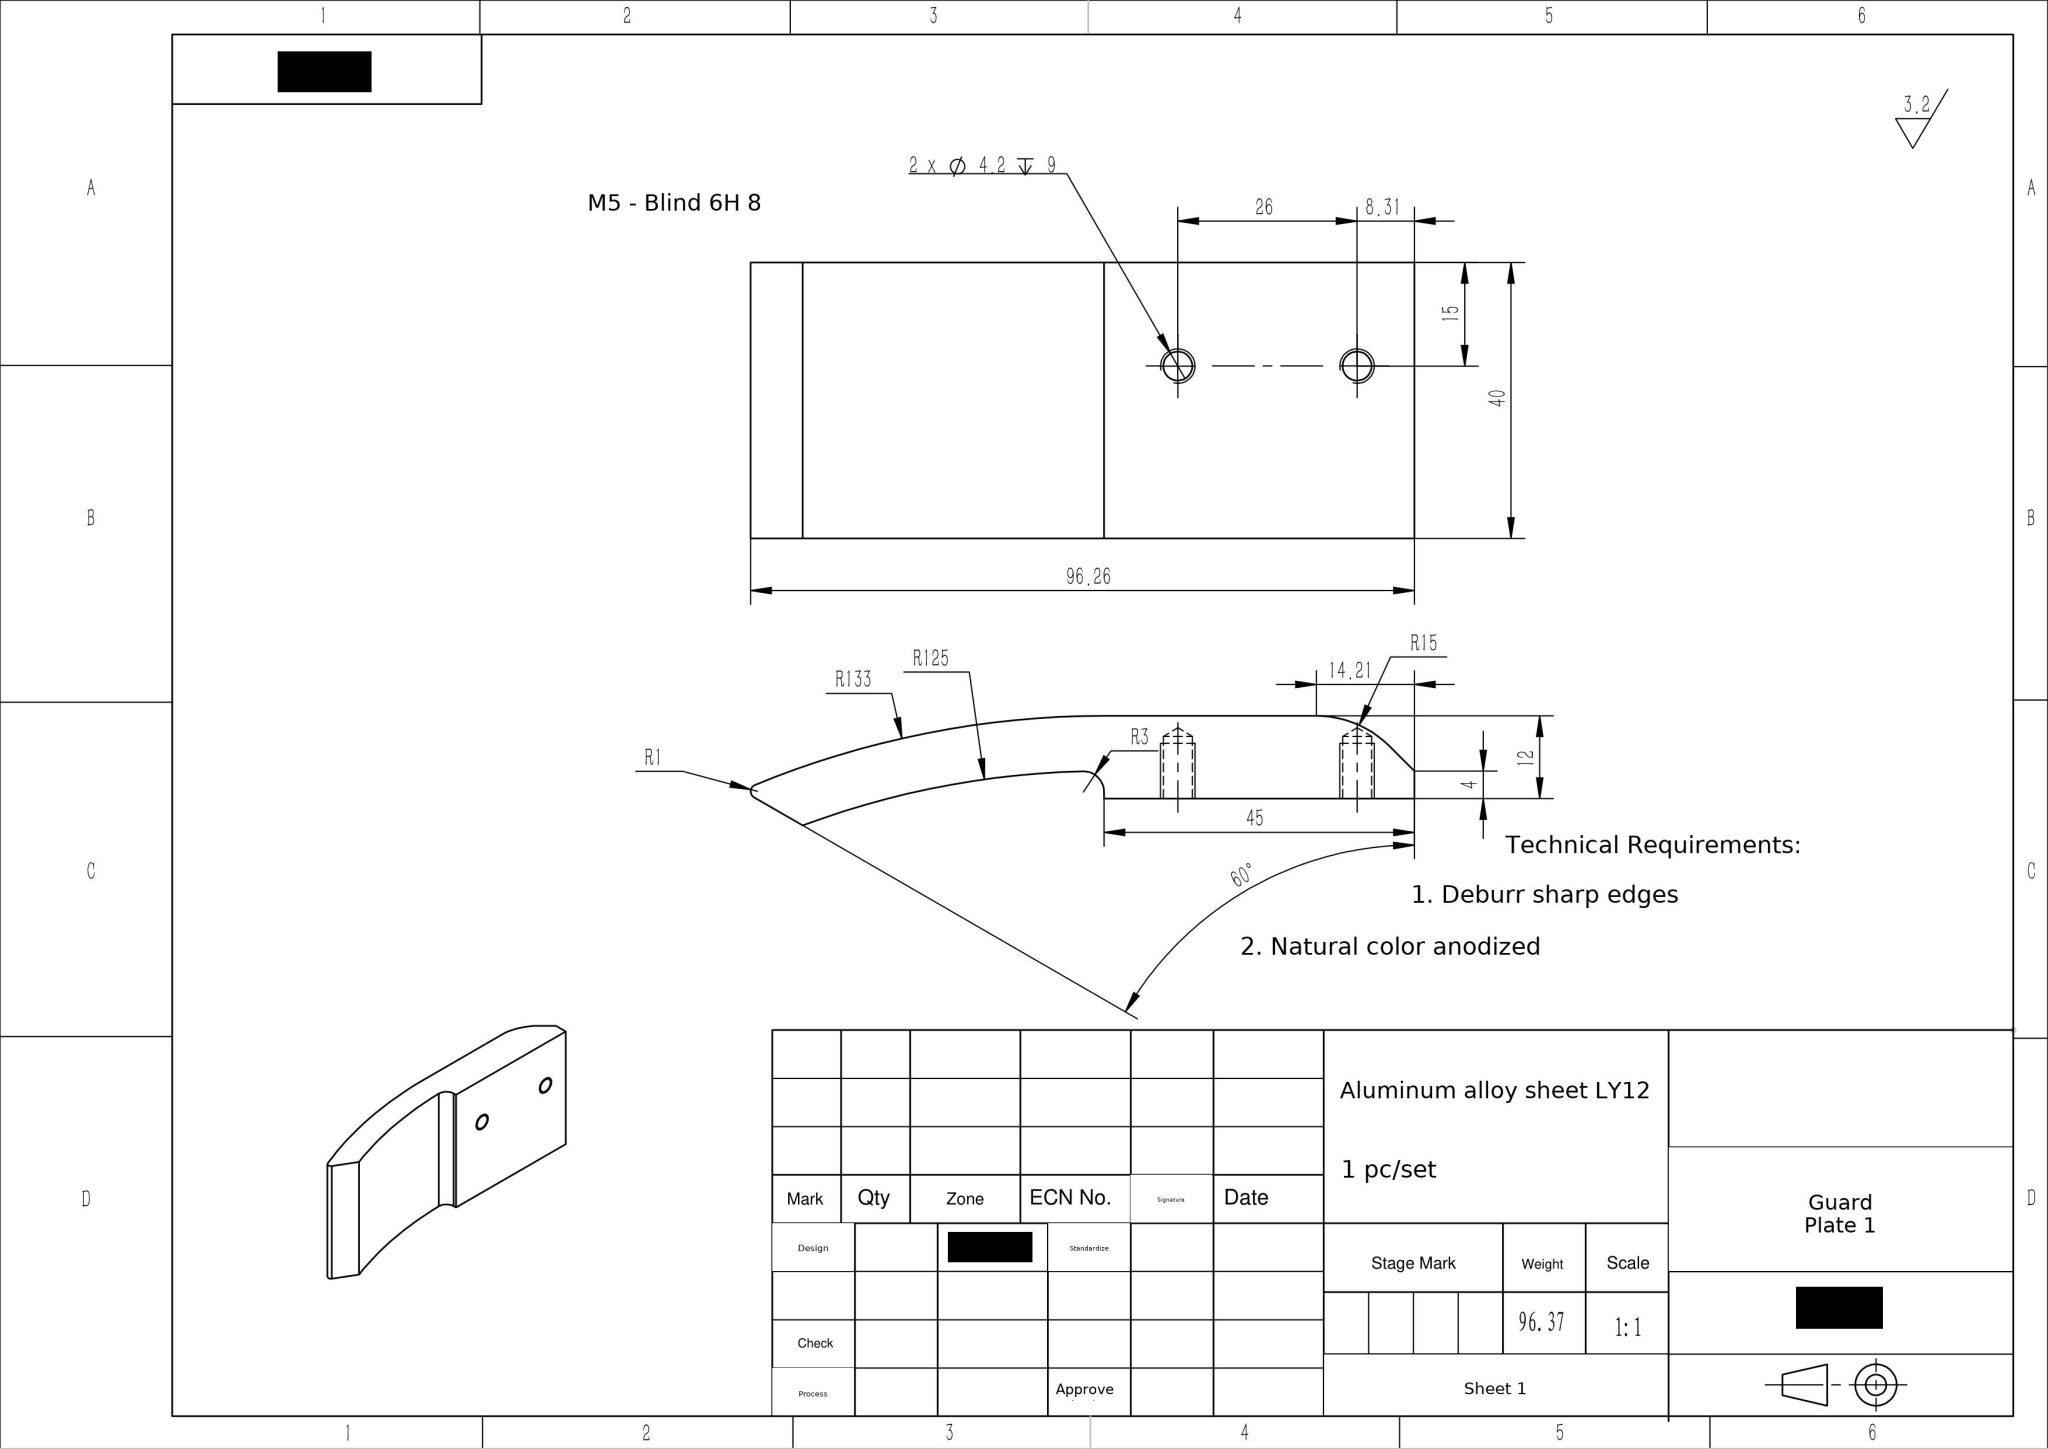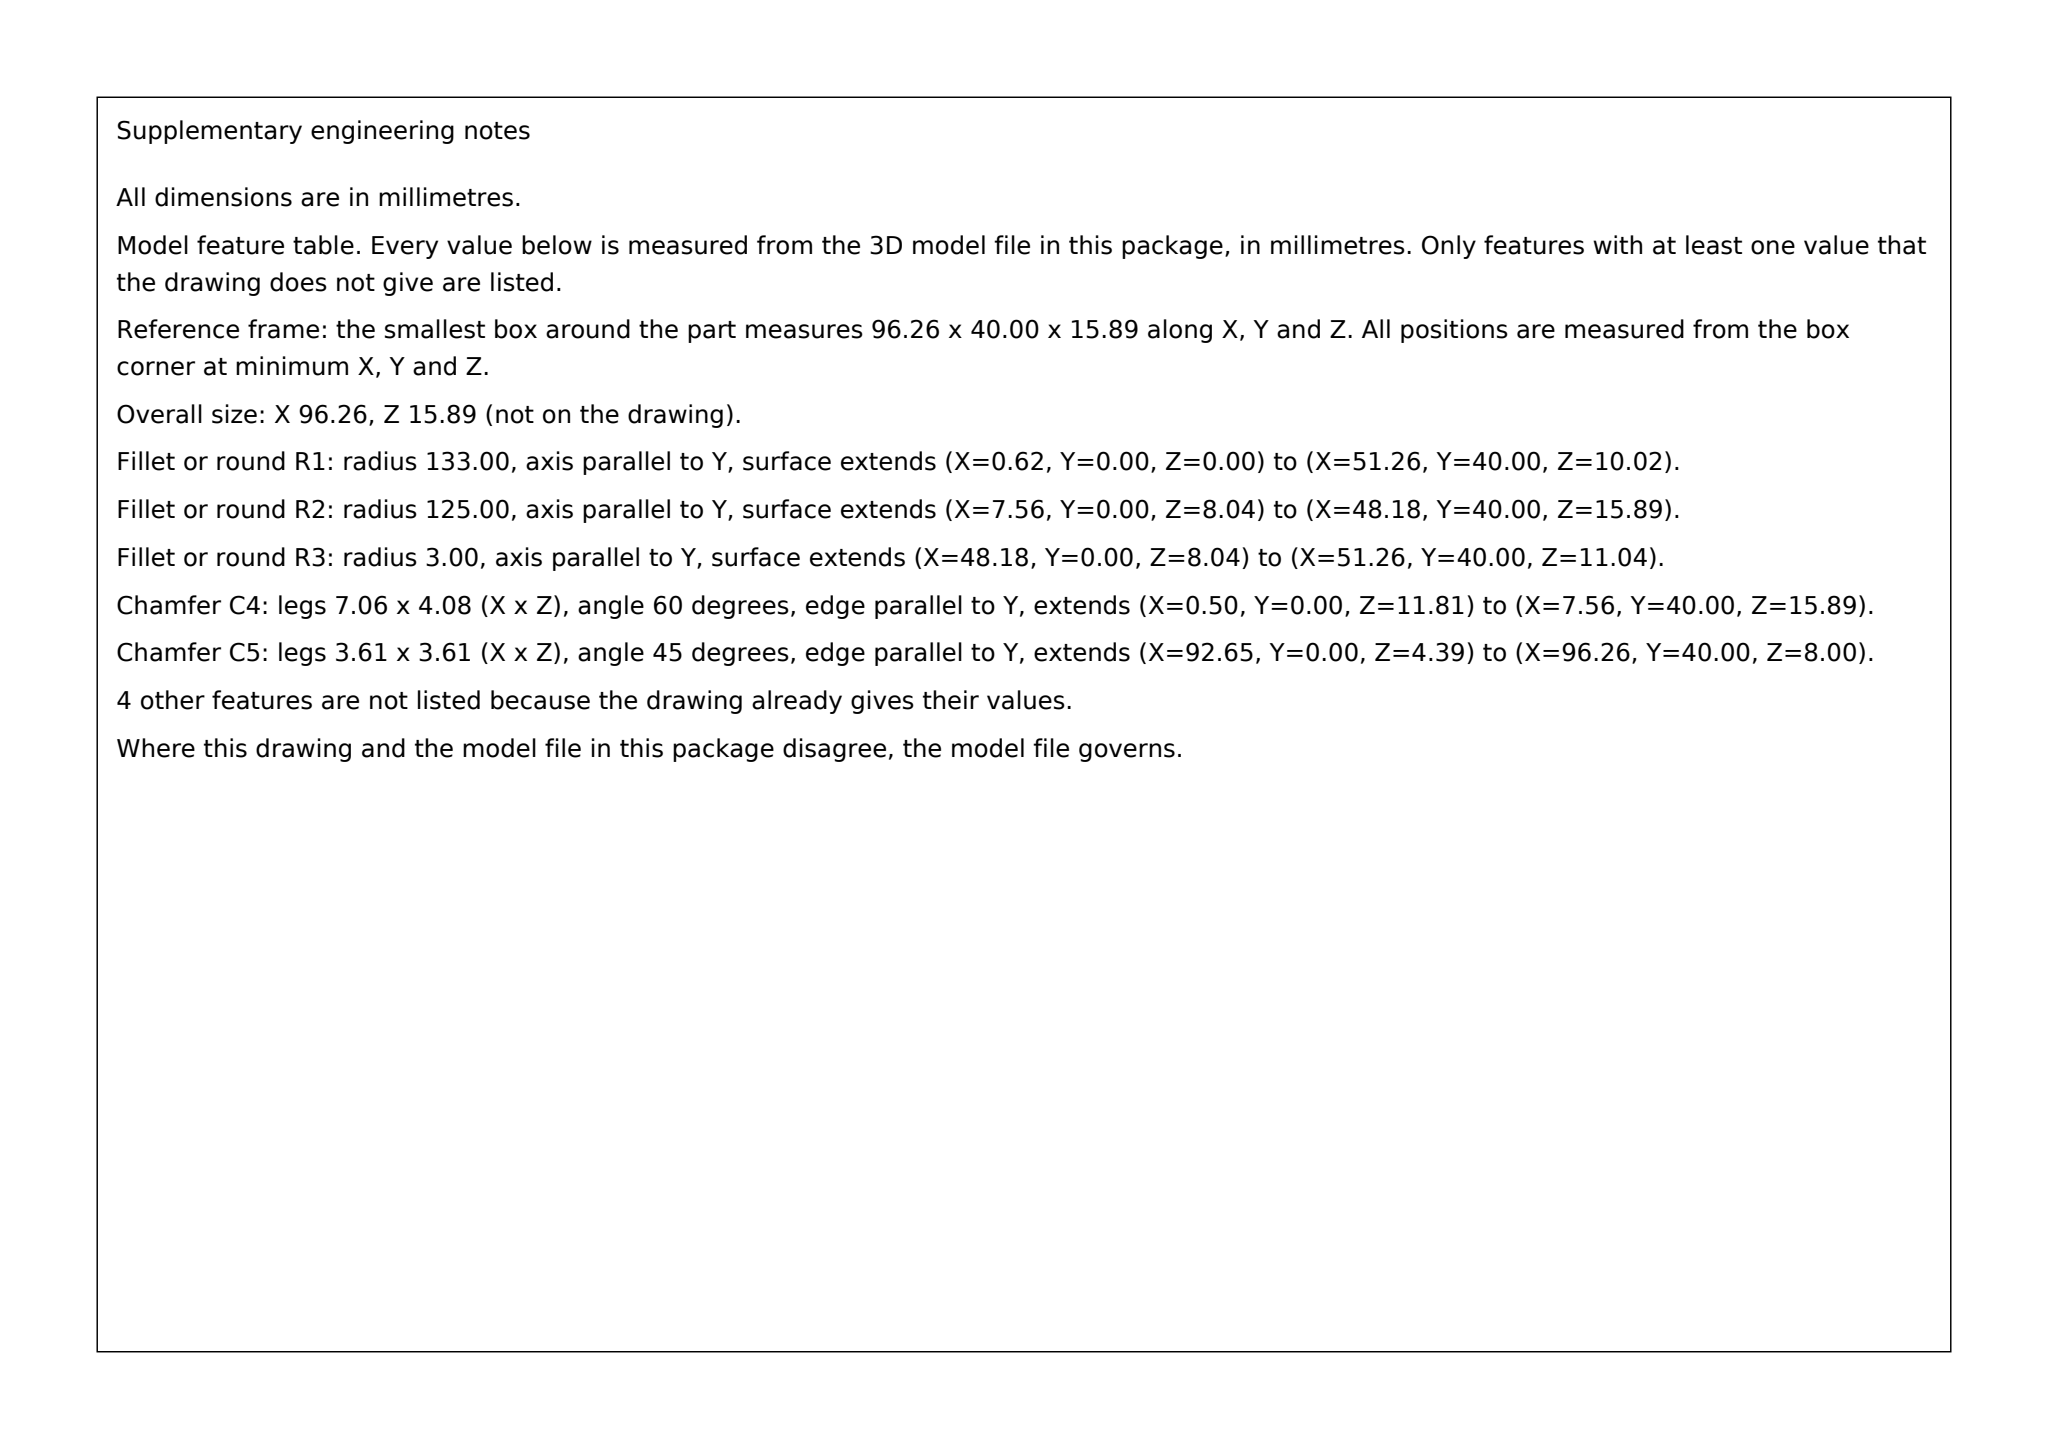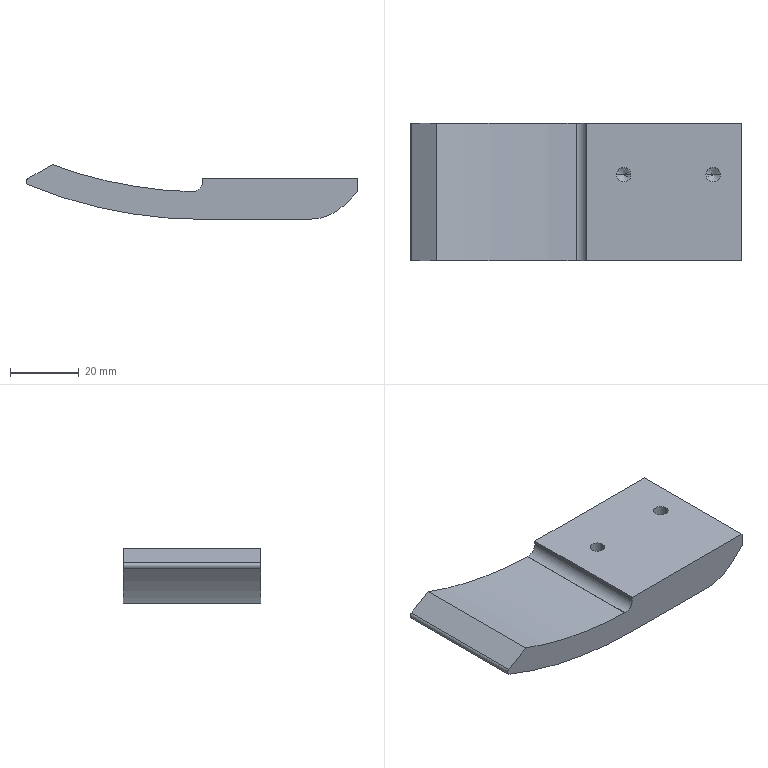Part | SolidWorks | mm | material Aluminum alloy sheet LY12 | 1 solid | 22 faces | box 96.26 x 40 x 15.89 mm | volume 35692 mm3 | cylinder 10 | plane 8 | cone 4 | commonest cylinder face diameters 4.2 x4 6 x2 250 x1 266 x1 30 x1 2 x1
build123d program:
from build123d import *

# Parameters (mm, degrees)
BOSS_EXTRUDE1_DEPTH   = 40
SKETCH5_W             = 45
SKETCH5_H             = 40
BOSS_EXTRUDE2_DEPTH   = 4
M5_TAPPED_HOLE1_D     = 4.2
M5_TAPPED_HOLE1_DEPTH = 9
M5_TAPPED_HOLE1_TIP   = 1.262
CHAMFER1_SIZE         = 8
FILLET1_R             = 15
FILLET2_R             = 1
FILLET3_R             = 3


with BuildPart() as part:
    # Sketch1 → Boss-Extrude1 (new body)
    with BuildSketch(Plane(origin=(0, 0, 0), x_dir=(1, 0, 0), z_dir=(0, 1, 0))):
        with BuildLine():
            Line((0, 0), (45, 0))
            Line((45, 0), (45, -8))
            Line((45, -8), (0, -8))
            ThreePointArc((0, -8), (-22.199, -9.987), (-43.693, -15.885))
            Line((-43.693, -15.885), (-52.5, -10.8))
            ThreePointArc((-52.5, -10.8), (-26.8, -2.728), (0, 0))
        make_face()
    extrude(amount=BOSS_EXTRUDE1_DEPTH)

    # Sketch5 → Boss-Extrude2 (add)
    with BuildSketch(Plane.XY.offset(8)):
        with Locations((22.5, 20)):
            Rectangle(SKETCH5_W, SKETCH5_H)
    extrude(amount=BOSS_EXTRUDE2_DEPTH)

    # M5 Tapped Hole1
    with Locations(Plane.XY.offset(12)):
        with Locations((36.695, 25), (10.695, 25)):
            Hole(M5_TAPPED_HOLE1_D / 2, depth=M5_TAPPED_HOLE1_DEPTH)
            with Locations((0, 0, -(M5_TAPPED_HOLE1_DEPTH + M5_TAPPED_HOLE1_TIP / 2))):  # 118° drill point
                Cone(0, M5_TAPPED_HOLE1_D / 2, M5_TAPPED_HOLE1_TIP, mode=Mode.SUBTRACT)

    # Chamfer1
    chamfer1_edges = [part.edges().sort_by_distance(p)[0] for p in [
        (45, 20, 0),
    ]]
    chamfer(chamfer1_edges, length=CHAMFER1_SIZE)

    # Fillet1
    fillet1_edges = [part.edges().sort_by_distance(p)[0] for p in [
        (37, 20, 0),
    ]]
    fillet(fillet1_edges, radius=FILLET1_R)

    # Fillet2
    fillet2_edges = [part.edges().sort_by_distance(p)[0] for p in [
        (-52.5, 20, 10.8),
    ]]
    fillet(fillet2_edges, radius=FILLET2_R)

    # Fillet3
    fillet3_edges = [part.edges().sort_by_distance(p)[0] for p in [
        (0, 20, 8),
    ]]
    fillet(fillet3_edges, radius=FILLET3_R)


solid = part.part
STEP:
#1=CARTESIAN_POINT('',(-3.,40.,8.037));
#2=VERTEX_POINT('',#1);
#3=CARTESIAN_POINT('',(0.,40.,11.037));
#4=VERTEX_POINT('',#3);
#5=CARTESIAN_POINT('',(-3.,40.,11.037));
#6=DIRECTION('',(0.,-1.,0.));
#7=DIRECTION('',(0.,0.,1.));
#8=AXIS2_PLACEMENT_3D('',#5,#6,#7);
#9=CIRCLE('',#8,3.);
#10=EDGE_CURVE('',#2,#4,#9,.T.);
#11=ORIENTED_EDGE('',*,*,#10,.F.);
#12=CARTESIAN_POINT('',(-3.,0.,8.037));
#13=VERTEX_POINT('',#12);
#14=CARTESIAN_POINT('',(-3.,40.,8.037));
#15=DIRECTION('',(0.,-1.,0.));
#16=VECTOR('',#15,1000.);
#17=LINE('',#14,#16);
#18=EDGE_CURVE('',#2,#13,#17,.T.);
#19=ORIENTED_EDGE('',*,*,#18,.T.);
#20=CARTESIAN_POINT('',(-0.,0.,11.037));
#21=VERTEX_POINT('',#20);
#22=CARTESIAN_POINT('',(-3.,0.,11.037));
#23=DIRECTION('',(0.,1.,0.));
#24=DIRECTION('',(0.,0.,1.));
#25=AXIS2_PLACEMENT_3D('',#22,#23,#24);
#26=CIRCLE('',#25,3.);
#27=EDGE_CURVE('',#21,#13,#26,.T.);
#28=ORIENTED_EDGE('',*,*,#27,.F.);
#29=CARTESIAN_POINT('',(-0.,-0.,11.037));
#30=DIRECTION('',(-0.,-1.,0.));
#31=VECTOR('',#30,1000.);
#32=LINE('',#29,#31);
#33=EDGE_CURVE('',#4,#21,#32,.T.);
#34=ORIENTED_EDGE('',*,*,#33,.F.);
#35=EDGE_LOOP('',(#11,#19,#28,#34));
#36=FACE_OUTER_BOUND('',#35,.T.);
#37=CARTESIAN_POINT('',(-3.,40.,11.037));
#38=DIRECTION('',(0.,-1.,0.));
#39=DIRECTION('',(0.,0.,-1.));
#40=AXIS2_PLACEMENT_3D('',#37,#38,#39);
#41=CYLINDRICAL_SURFACE('',#40,3.);
#42=ADVANCED_FACE('',(#36),#41,.F.);
#43=CARTESIAN_POINT('',(34.595,25.,3.));
#44=VERTEX_POINT('',#43);
#45=CARTESIAN_POINT('',(38.795,25.,3.));
#46=VERTEX_POINT('',#45);
#47=CARTESIAN_POINT('',(36.695,25.,3.));
#48=DIRECTION('',(0.,0.,1.));
#49=DIRECTION('',(1.,0.,0.));
#50=AXIS2_PLACEMENT_3D('',#47,#48,#49);
#51=CIRCLE('',#50,2.1);
#52=EDGE_CURVE('',#44,#46,#51,.T.);
#53=ORIENTED_EDGE('',*,*,#52,.F.);
#54=CARTESIAN_POINT('',(34.595,25.,12.));
#55=VERTEX_POINT('',#54);
#56=CARTESIAN_POINT('',(34.595,25.,12.));
#57=DIRECTION('',(0.,0.,1.));
#58=VECTOR('',#57,1000.);
#59=LINE('',#56,#58);
#60=EDGE_CURVE('',#44,#55,#59,.T.);
#61=ORIENTED_EDGE('',*,*,#60,.T.);
#62=CARTESIAN_POINT('',(38.795,25.,12.));
#63=VERTEX_POINT('',#62);
#64=CARTESIAN_POINT('',(36.695,25.,12.));
#65=DIRECTION('',(0.,0.,1.));
#66=DIRECTION('',(1.,0.,0.));
#67=AXIS2_PLACEMENT_3D('',#64,#65,#66);
#68=CIRCLE('',#67,2.1);
#69=EDGE_CURVE('',#55,#63,#68,.T.);
#70=ORIENTED_EDGE('',*,*,#69,.T.);
#71=CARTESIAN_POINT('',(38.795,25.,12.));
#72=DIRECTION('',(0.,0.,1.));
#73=VECTOR('',#72,1000.);
#74=LINE('',#71,#73);
#75=EDGE_CURVE('',#46,#63,#74,.T.);
#76=ORIENTED_EDGE('',*,*,#75,.F.);
#77=EDGE_LOOP('',(#53,#61,#70,#76));
#78=FACE_OUTER_BOUND('',#77,.T.);
#79=CARTESIAN_POINT('',(36.695,25.,12.));
#80=DIRECTION('',(0.,0.,1.));
#81=DIRECTION('',(1.,0.,0.));
#82=AXIS2_PLACEMENT_3D('',#79,#80,#81);
#83=CYLINDRICAL_SURFACE('',#82,2.1);
#84=ADVANCED_FACE('',(#78),#83,.F.);
#85=CARTESIAN_POINT('',(36.695,25.,1.738));
#86=VERTEX_POINT('',#85);
#87=CARTESIAN_POINT('',(38.795,25.,3.));
#88=DIRECTION('',(0.8572,0.,0.515));
#89=VECTOR('',#88,1000.);
#90=LINE('',#87,#89);
#91=EDGE_CURVE('',#86,#46,#90,.T.);
#92=ORIENTED_EDGE('',*,*,#91,.F.);
#93=CARTESIAN_POINT('',(34.595,25.,3.));
#94=DIRECTION('',(-0.8572,0.,0.515));
#95=VECTOR('',#94,1000.);
#96=LINE('',#93,#95);
#97=EDGE_CURVE('',#86,#44,#96,.T.);
#98=ORIENTED_EDGE('',*,*,#97,.T.);
#99=ORIENTED_EDGE('',*,*,#52,.T.);
#100=EDGE_LOOP('',(#92,#98,#99));
#101=FACE_OUTER_BOUND('',#100,.T.);
#102=CARTESIAN_POINT('',(36.695,25.,3.));
#103=DIRECTION('',(0.,0.,1.));
#104=DIRECTION('',(1.,0.,0.));
#105=AXIS2_PLACEMENT_3D('',#102,#103,#104);
#106=CONICAL_SURFACE('',#105,2.1,1.03);
#107=ADVANCED_FACE('',(#101),#106,.F.);
#108=CARTESIAN_POINT('',(8.595,25.,3.));
#109=VERTEX_POINT('',#108);
#110=CARTESIAN_POINT('',(12.795,25.,3.));
#111=VERTEX_POINT('',#110);
#112=CARTESIAN_POINT('',(10.695,25.,3.));
#113=DIRECTION('',(0.,0.,1.));
#114=DIRECTION('',(1.,0.,0.));
#115=AXIS2_PLACEMENT_3D('',#112,#113,#114);
#116=CIRCLE('',#115,2.1);
#117=EDGE_CURVE('',#109,#111,#116,.T.);
#118=ORIENTED_EDGE('',*,*,#117,.F.);
#119=CARTESIAN_POINT('',(8.595,25.,12.));
#120=VERTEX_POINT('',#119);
#121=CARTESIAN_POINT('',(8.595,25.,12.));
#122=DIRECTION('',(0.,0.,1.));
#123=VECTOR('',#122,1000.);
#124=LINE('',#121,#123);
#125=EDGE_CURVE('',#109,#120,#124,.T.);
#126=ORIENTED_EDGE('',*,*,#125,.T.);
#127=CARTESIAN_POINT('',(12.795,25.,12.));
#128=VERTEX_POINT('',#127);
#129=CARTESIAN_POINT('',(10.695,25.,12.));
#130=DIRECTION('',(0.,0.,1.));
#131=DIRECTION('',(1.,0.,0.));
#132=AXIS2_PLACEMENT_3D('',#129,#130,#131);
#133=CIRCLE('',#132,2.1);
#134=EDGE_CURVE('',#120,#128,#133,.T.);
#135=ORIENTED_EDGE('',*,*,#134,.T.);
#136=CARTESIAN_POINT('',(12.795,25.,12.));
#137=DIRECTION('',(0.,0.,1.));
#138=VECTOR('',#137,1000.);
#139=LINE('',#136,#138);
#140=EDGE_CURVE('',#111,#128,#139,.T.);
#141=ORIENTED_EDGE('',*,*,#140,.F.);
#142=EDGE_LOOP('',(#118,#126,#135,#141));
#143=FACE_OUTER_BOUND('',#142,.T.);
#144=CARTESIAN_POINT('',(10.695,25.,12.));
#145=DIRECTION('',(0.,0.,1.));
#146=DIRECTION('',(1.,0.,0.));
#147=AXIS2_PLACEMENT_3D('',#144,#145,#146);
#148=CYLINDRICAL_SURFACE('',#147,2.1);
#149=ADVANCED_FACE('',(#143),#148,.F.);
#150=CARTESIAN_POINT('',(10.695,25.,1.738));
#151=VERTEX_POINT('',#150);
#152=CARTESIAN_POINT('',(12.795,25.,3.));
#153=DIRECTION('',(0.8572,0.,0.515));
#154=VECTOR('',#153,1000.);
#155=LINE('',#152,#154);
#156=EDGE_CURVE('',#151,#111,#155,.T.);
#157=ORIENTED_EDGE('',*,*,#156,.F.);
#158=CARTESIAN_POINT('',(8.595,25.,3.));
#159=DIRECTION('',(-0.8572,0.,0.515));
#160=VECTOR('',#159,1000.);
#161=LINE('',#158,#160);
#162=EDGE_CURVE('',#151,#109,#161,.T.);
#163=ORIENTED_EDGE('',*,*,#162,.T.);
#164=ORIENTED_EDGE('',*,*,#117,.T.);
#165=EDGE_LOOP('',(#157,#163,#164));
#166=FACE_OUTER_BOUND('',#165,.T.);
#167=CARTESIAN_POINT('',(10.695,25.,3.));
#168=DIRECTION('',(0.,0.,1.));
#169=DIRECTION('',(1.,0.,0.));
#170=AXIS2_PLACEMENT_3D('',#167,#168,#169);
#171=CONICAL_SURFACE('',#170,2.1,1.03);
#172=ADVANCED_FACE('',(#166),#171,.F.);
#173=CARTESIAN_POINT('',(-43.693,0.,15.885));
#174=VERTEX_POINT('',#173);
#175=CARTESIAN_POINT('',(-3.074,0.,8.038));
#176=VERTEX_POINT('',#175);
#177=CARTESIAN_POINT('',(0.,0.,133.));
#178=DIRECTION('',(0.,-1.,0.));
#179=DIRECTION('',(0.,0.,1.));
#180=AXIS2_PLACEMENT_3D('',#177,#178,#179);
#181=CIRCLE('',#180,125.);
#182=EDGE_CURVE('',#174,#176,#181,.T.);
#183=ORIENTED_EDGE('',*,*,#182,.T.);
#184=CARTESIAN_POINT('',(-3.074,40.,8.038));
#185=VERTEX_POINT('',#184);
#186=CARTESIAN_POINT('',(-3.074,40.,8.038));
#187=DIRECTION('',(0.,1.,0.));
#188=VECTOR('',#187,1000.);
#189=LINE('',#186,#188);
#190=EDGE_CURVE('',#176,#185,#189,.T.);
#191=ORIENTED_EDGE('',*,*,#190,.T.);
#192=CARTESIAN_POINT('',(-43.693,40.,15.885));
#193=VERTEX_POINT('',#192);
#194=CARTESIAN_POINT('',(0.,40.,133.));
#195=DIRECTION('',(0.,-1.,0.));
#196=DIRECTION('',(0.,0.,1.));
#197=AXIS2_PLACEMENT_3D('',#194,#195,#196);
#198=CIRCLE('',#197,125.);
#199=EDGE_CURVE('',#193,#185,#198,.T.);
#200=ORIENTED_EDGE('',*,*,#199,.F.);
#201=CARTESIAN_POINT('',(-43.693,40.,15.885));
#202=DIRECTION('',(0.,-1.,0.));
#203=VECTOR('',#202,1000.);
#204=LINE('',#201,#203);
#205=EDGE_CURVE('',#193,#174,#204,.T.);
#206=ORIENTED_EDGE('',*,*,#205,.T.);
#207=EDGE_LOOP('',(#183,#191,#200,#206));
#208=FACE_OUTER_BOUND('',#207,.T.);
#209=CARTESIAN_POINT('',(0.,40.,133.));
#210=DIRECTION('',(0.,-1.,0.));
#211=DIRECTION('',(0.,0.,-1.));
#212=AXIS2_PLACEMENT_3D('',#209,#210,#211);
#213=CYLINDRICAL_SURFACE('',#212,125.);
#214=ADVANCED_FACE('',(#208),#213,.F.);
#215=CARTESIAN_POINT('',(45.,-0.,12.));
#216=VERTEX_POINT('',#215);
#217=CARTESIAN_POINT('',(45.,0.,8.));
#218=VERTEX_POINT('',#217);
#219=CARTESIAN_POINT('',(45.,0.,0.));
#220=DIRECTION('',(0.,0.,-1.));
#221=VECTOR('',#220,1000.);
#222=LINE('',#219,#221);
#223=EDGE_CURVE('',#216,#218,#222,.T.);
#224=ORIENTED_EDGE('',*,*,#223,.T.);
#225=CARTESIAN_POINT('',(45.,40.,8.));
#226=VERTEX_POINT('',#225);
#227=CARTESIAN_POINT('',(45.,40.,8.));
#228=DIRECTION('',(0.,1.,0.));
#229=VECTOR('',#228,1000.);
#230=LINE('',#227,#229);
#231=EDGE_CURVE('',#218,#226,#230,.T.);
#232=ORIENTED_EDGE('',*,*,#231,.T.);
#233=CARTESIAN_POINT('',(45.,40.,12.));
#234=VERTEX_POINT('',#233);
#235=CARTESIAN_POINT('',(45.,40.,0.));
#236=DIRECTION('',(0.,0.,-1.));
#237=VECTOR('',#236,1000.);
#238=LINE('',#235,#237);
#239=EDGE_CURVE('',#234,#226,#238,.T.);
#240=ORIENTED_EDGE('',*,*,#239,.F.);
#241=CARTESIAN_POINT('',(45.,40.,12.));
#242=DIRECTION('',(-0.,1.,0.));
#243=VECTOR('',#242,1000.);
#244=LINE('',#241,#243);
#245=EDGE_CURVE('',#216,#234,#244,.T.);
#246=ORIENTED_EDGE('',*,*,#245,.F.);
#247=EDGE_LOOP('',(#224,#232,#240,#246));
#248=FACE_OUTER_BOUND('',#247,.T.);
#249=CARTESIAN_POINT('',(45.,40.,0.));
#250=DIRECTION('',(-1.,0.,0.));
#251=DIRECTION('',(0.,0.,1.));
#252=AXIS2_PLACEMENT_3D('',#249,#250,#251);
#253=PLANE('',#252);
#254=ADVANCED_FACE('',(#248),#253,.F.);
#255=CARTESIAN_POINT('',(30.787,40.,0.));
#256=VERTEX_POINT('',#255);
#257=CARTESIAN_POINT('',(0.,40.,0.));
#258=VERTEX_POINT('',#257);
#259=CARTESIAN_POINT('',(0.,40.,0.));
#260=DIRECTION('',(-1.,0.,0.));
#261=VECTOR('',#260,1000.);
#262=LINE('',#259,#261);
#263=EDGE_CURVE('',#256,#258,#262,.T.);
#264=ORIENTED_EDGE('',*,*,#263,.F.);
#265=CARTESIAN_POINT('',(30.787,0.,0.));
#266=VERTEX_POINT('',#265);
#267=CARTESIAN_POINT('',(30.787,0.,0.));
#268=DIRECTION('',(0.,-1.,0.));
#269=VECTOR('',#268,1000.);
#270=LINE('',#267,#269);
#271=EDGE_CURVE('',#256,#266,#270,.T.);
#272=ORIENTED_EDGE('',*,*,#271,.T.);
#273=CARTESIAN_POINT('',(0.,0.,0.));
#274=VERTEX_POINT('',#273);
#275=CARTESIAN_POINT('',(0.,0.,0.));
#276=DIRECTION('',(-1.,0.,0.));
#277=VECTOR('',#276,1000.);
#278=LINE('',#275,#277);
#279=EDGE_CURVE('',#266,#274,#278,.T.);
#280=ORIENTED_EDGE('',*,*,#279,.T.);
#281=CARTESIAN_POINT('',(0.,40.,0.));
#282=DIRECTION('',(0.,-1.,0.));
#283=VECTOR('',#282,1000.);
#284=LINE('',#281,#283);
#285=EDGE_CURVE('',#258,#274,#284,.T.);
#286=ORIENTED_EDGE('',*,*,#285,.F.);
#287=EDGE_LOOP('',(#264,#272,#280,#286));
#288=FACE_OUTER_BOUND('',#287,.T.);
#289=CARTESIAN_POINT('',(0.,40.,0.));
#290=DIRECTION('',(0.,0.,1.));
#291=DIRECTION('',(1.,0.,0.));
#292=AXIS2_PLACEMENT_3D('',#289,#290,#291);
#293=PLANE('',#292);
#294=ADVANCED_FACE('',(#288),#293,.F.);
#295=CARTESIAN_POINT('',(-50.637,0.,10.017));
#296=VERTEX_POINT('',#295);
#297=CARTESIAN_POINT('',(0.,0.,133.));
#298=DIRECTION('',(0.,1.,0.));
#299=DIRECTION('',(0.,0.,1.));
#300=AXIS2_PLACEMENT_3D('',#297,#298,#299);
#301=CIRCLE('',#300,133.);
#302=EDGE_CURVE('',#274,#296,#301,.T.);
#303=ORIENTED_EDGE('',*,*,#302,.T.);
#304=CARTESIAN_POINT('',(-50.637,40.,10.017));
#305=VERTEX_POINT('',#304);
#306=CARTESIAN_POINT('',(-50.637,40.,10.017));
#307=DIRECTION('',(0.,1.,0.));
#308=VECTOR('',#307,1000.);
#309=LINE('',#306,#308);
#310=EDGE_CURVE('',#296,#305,#309,.T.);
#311=ORIENTED_EDGE('',*,*,#310,.T.);
#312=CARTESIAN_POINT('',(0.,40.,133.));
#313=DIRECTION('',(0.,1.,0.));
#314=DIRECTION('',(0.,0.,1.));
#315=AXIS2_PLACEMENT_3D('',#312,#313,#314);
#316=CIRCLE('',#315,133.);
#317=EDGE_CURVE('',#258,#305,#316,.T.);
#318=ORIENTED_EDGE('',*,*,#317,.F.);
#319=ORIENTED_EDGE('',*,*,#285,.T.);
#320=EDGE_LOOP('',(#303,#311,#318,#319));
#321=FACE_OUTER_BOUND('',#320,.T.);
#322=CARTESIAN_POINT('',(0.,40.,133.));
#323=DIRECTION('',(0.,-1.,0.));
#324=DIRECTION('',(0.,0.,-1.));
#325=AXIS2_PLACEMENT_3D('',#322,#323,#324);
#326=CYLINDRICAL_SURFACE('',#325,133.);
#327=ADVANCED_FACE('',(#321),#326,.T.);
#328=CARTESIAN_POINT('',(-50.756,40.,11.807));
#329=VERTEX_POINT('',#328);
#330=CARTESIAN_POINT('',(-43.693,40.,15.885));
#331=DIRECTION('',(0.866,0.,0.5));
#332=VECTOR('',#331,1000.);
#333=LINE('',#330,#332);
#334=EDGE_CURVE('',#329,#193,#333,.T.);
#335=ORIENTED_EDGE('',*,*,#334,.F.);
#336=CARTESIAN_POINT('',(-50.756,0.,11.807));
#337=VERTEX_POINT('',#336);
#338=CARTESIAN_POINT('',(-50.756,40.,11.807));
#339=DIRECTION('',(0.,-1.,0.));
#340=VECTOR('',#339,1000.);
#341=LINE('',#338,#340);
#342=EDGE_CURVE('',#329,#337,#341,.T.);
#343=ORIENTED_EDGE('',*,*,#342,.T.);
#344=CARTESIAN_POINT('',(-43.693,0.,15.885));
#345=DIRECTION('',(0.866,0.,0.5));
#346=VECTOR('',#345,1000.);
#347=LINE('',#344,#346);
#348=EDGE_CURVE('',#337,#174,#347,.T.);
#349=ORIENTED_EDGE('',*,*,#348,.T.);
#350=ORIENTED_EDGE('',*,*,#205,.F.);
#351=EDGE_LOOP('',(#335,#343,#349,#350));
#352=FACE_OUTER_BOUND('',#351,.T.);
#353=CARTESIAN_POINT('',(-43.693,40.,15.885));
#354=DIRECTION('',(0.5,0.,-0.866));
#355=DIRECTION('',(-0.866,0.,-0.5));
#356=AXIS2_PLACEMENT_3D('',#353,#354,#355);
#357=PLANE('',#356);
#358=ADVANCED_FACE('',(#352),#357,.F.);
#359=ORIENTED_EDGE('',*,*,#317,.T.);
#360=CARTESIAN_POINT('',(-50.256,40.,10.941));
#361=DIRECTION('',(0.,1.,0.));
#362=DIRECTION('',(0.,0.,1.));
#363=AXIS2_PLACEMENT_3D('',#360,#361,#362);
#364=CIRCLE('',#363,1.);
#365=EDGE_CURVE('',#305,#329,#364,.T.);
#366=ORIENTED_EDGE('',*,*,#365,.T.);
#367=ORIENTED_EDGE('',*,*,#334,.T.);
#368=ORIENTED_EDGE('',*,*,#199,.T.);
#369=CARTESIAN_POINT('',(-3.,40.,11.037));
#370=DIRECTION('',(0.,-1.,0.));
#371=DIRECTION('',(0.,0.,1.));
#372=AXIS2_PLACEMENT_3D('',#369,#370,#371);
#373=CIRCLE('',#372,3.);
#374=EDGE_CURVE('',#185,#2,#373,.T.);
#375=ORIENTED_EDGE('',*,*,#374,.T.);
#376=ORIENTED_EDGE('',*,*,#10,.T.);
#377=CARTESIAN_POINT('',(0.,40.,12.));
#378=VERTEX_POINT('',#377);
#379=CARTESIAN_POINT('',(0.,40.,12.));
#380=DIRECTION('',(0.,0.,-1.));
#381=VECTOR('',#380,1000.);
#382=LINE('',#379,#381);
#383=EDGE_CURVE('',#378,#4,#382,.T.);
#384=ORIENTED_EDGE('',*,*,#383,.F.);
#385=CARTESIAN_POINT('',(45.,40.,12.));
#386=DIRECTION('',(-1.,-0.,0.));
#387=VECTOR('',#386,1000.);
#388=LINE('',#385,#387);
#389=EDGE_CURVE('',#234,#378,#388,.T.);
#390=ORIENTED_EDGE('',*,*,#389,.F.);
#391=ORIENTED_EDGE('',*,*,#239,.T.);
#392=CARTESIAN_POINT('',(41.393,40.,4.393));
#393=VERTEX_POINT('',#392);
#394=CARTESIAN_POINT('',(85.,40.,48.));
#395=DIRECTION('',(-0.7071,0.,-0.7071));
#396=VECTOR('',#395,1000.);
#397=LINE('',#394,#396);
#398=EDGE_CURVE('',#226,#393,#397,.T.);
#399=ORIENTED_EDGE('',*,*,#398,.T.);
#400=CARTESIAN_POINT('',(30.787,40.,15.));
#401=DIRECTION('',(0.,1.,0.));
#402=DIRECTION('',(0.,0.,1.));
#403=AXIS2_PLACEMENT_3D('',#400,#401,#402);
#404=CIRCLE('',#403,15.);
#405=EDGE_CURVE('',#393,#256,#404,.T.);
#406=ORIENTED_EDGE('',*,*,#405,.T.);
#407=ORIENTED_EDGE('',*,*,#263,.T.);
#408=EDGE_LOOP('',(#359,#366,#367,#368,#375,#376,#384,#390,#391,#399,#406,#407));
#409=FACE_OUTER_BOUND('',#408,.T.);
#410=CARTESIAN_POINT('',(0.,40.,133.));
#411=DIRECTION('',(0.,1.,0.));
#412=DIRECTION('',(0.,0.,1.));
#413=AXIS2_PLACEMENT_3D('',#410,#411,#412);
#414=PLANE('',#413);
#415=ADVANCED_FACE('',(#409),#414,.T.);
#416=ORIENTED_EDGE('',*,*,#348,.F.);
#417=CARTESIAN_POINT('',(-50.256,0.,10.941));
#418=DIRECTION('',(0.,-1.,0.));
#419=DIRECTION('',(-0.,0.,1.));
#420=AXIS2_PLACEMENT_3D('',#417,#418,#419);
#421=CIRCLE('',#420,1.);
#422=EDGE_CURVE('',#337,#296,#421,.T.);
#423=ORIENTED_EDGE('',*,*,#422,.T.);
#424=ORIENTED_EDGE('',*,*,#302,.F.);
#425=ORIENTED_EDGE('',*,*,#279,.F.);
#426=CARTESIAN_POINT('',(41.393,0.,4.393));
#427=VERTEX_POINT('',#426);
#428=CARTESIAN_POINT('',(30.787,0.,15.));
#429=DIRECTION('',(0.,-1.,0.));
#430=DIRECTION('',(0.,0.,1.));
#431=AXIS2_PLACEMENT_3D('',#428,#429,#430);
#432=CIRCLE('',#431,15.);
#433=EDGE_CURVE('',#266,#427,#432,.T.);
#434=ORIENTED_EDGE('',*,*,#433,.T.);
#435=CARTESIAN_POINT('',(37.,0.,0.));
#436=DIRECTION('',(0.7071,0.,0.7071));
#437=VECTOR('',#436,1000.);
#438=LINE('',#435,#437);
#439=EDGE_CURVE('',#427,#218,#438,.T.);
#440=ORIENTED_EDGE('',*,*,#439,.T.);
#441=ORIENTED_EDGE('',*,*,#223,.F.);
#442=CARTESIAN_POINT('',(-0.,0.,12.));
#443=VERTEX_POINT('',#442);
#444=CARTESIAN_POINT('',(45.,-0.,12.));
#445=DIRECTION('',(1.,-0.,0.));
#446=VECTOR('',#445,1000.);
#447=LINE('',#444,#446);
#448=EDGE_CURVE('',#443,#216,#447,.T.);
#449=ORIENTED_EDGE('',*,*,#448,.F.);
#450=CARTESIAN_POINT('',(-0.,0.,12.));
#451=DIRECTION('',(0.,0.,-1.));
#452=VECTOR('',#451,1000.);
#453=LINE('',#450,#452);
#454=EDGE_CURVE('',#443,#21,#453,.T.);
#455=ORIENTED_EDGE('',*,*,#454,.T.);
#456=ORIENTED_EDGE('',*,*,#27,.T.);
#457=CARTESIAN_POINT('',(-3.,0.,11.037));
#458=DIRECTION('',(0.,1.,0.));
#459=DIRECTION('',(0.,0.,1.));
#460=AXIS2_PLACEMENT_3D('',#457,#458,#459);
#461=CIRCLE('',#460,3.);
#462=EDGE_CURVE('',#13,#176,#461,.T.);
#463=ORIENTED_EDGE('',*,*,#462,.T.);
#464=ORIENTED_EDGE('',*,*,#182,.F.);
#465=EDGE_LOOP('',(#416,#423,#424,#425,#434,#440,#441,#449,#455,#456,#463,#464));
#466=FACE_OUTER_BOUND('',#465,.T.);
#467=CARTESIAN_POINT('',(0.,0.,133.));
#468=DIRECTION('',(0.,1.,0.));
#469=DIRECTION('',(0.,0.,1.));
#470=AXIS2_PLACEMENT_3D('',#467,#468,#469);
#471=PLANE('',#470);
#472=ADVANCED_FACE('',(#466),#471,.F.);
#473=ORIENTED_EDGE('',*,*,#383,.T.);
#474=ORIENTED_EDGE('',*,*,#33,.T.);
#475=ORIENTED_EDGE('',*,*,#454,.F.);
#476=CARTESIAN_POINT('',(0.,40.,12.));
#477=DIRECTION('',(-0.,-1.,0.));
#478=VECTOR('',#477,1000.);
#479=LINE('',#476,#478);
#480=EDGE_CURVE('',#378,#443,#479,.T.);
#481=ORIENTED_EDGE('',*,*,#480,.F.);
#482=EDGE_LOOP('',(#473,#474,#475,#481));
#483=FACE_OUTER_BOUND('',#482,.T.);
#484=CARTESIAN_POINT('',(0.,40.,12.));
#485=DIRECTION('',(1.,-0.,0.));
#486=DIRECTION('',(0.,1.,0.));
#487=AXIS2_PLACEMENT_3D('',#484,#485,#486);
#488=PLANE('',#487);
#489=ADVANCED_FACE('',(#483),#488,.F.);
#490=CARTESIAN_POINT('',(36.695,25.,12.));
#491=DIRECTION('',(0.,0.,1.));
#492=DIRECTION('',(1.,0.,0.));
#493=AXIS2_PLACEMENT_3D('',#490,#491,#492);
#494=CIRCLE('',#493,2.1);
#495=EDGE_CURVE('',#63,#55,#494,.T.);
#496=ORIENTED_EDGE('',*,*,#495,.F.);
#497=ORIENTED_EDGE('',*,*,#69,.F.);
#498=EDGE_LOOP('',(#496,#497));
#499=FACE_BOUND('',#498,.T.);
#500=CARTESIAN_POINT('',(10.695,25.,12.));
#501=DIRECTION('',(0.,0.,1.));
#502=DIRECTION('',(1.,0.,0.));
#503=AXIS2_PLACEMENT_3D('',#500,#501,#502);
#504=CIRCLE('',#503,2.1);
#505=EDGE_CURVE('',#128,#120,#504,.T.);
#506=ORIENTED_EDGE('',*,*,#505,.F.);
#507=ORIENTED_EDGE('',*,*,#134,.F.);
#508=EDGE_LOOP('',(#506,#507));
#509=FACE_BOUND('',#508,.T.);
#510=ORIENTED_EDGE('',*,*,#245,.T.);
#511=ORIENTED_EDGE('',*,*,#389,.T.);
#512=ORIENTED_EDGE('',*,*,#480,.T.);
#513=ORIENTED_EDGE('',*,*,#448,.T.);
#514=EDGE_LOOP('',(#510,#511,#512,#513));
#515=FACE_OUTER_BOUND('',#514,.T.);
#516=CARTESIAN_POINT('',(0.,0.,12.));
#517=DIRECTION('',(0.,0.,-1.));
#518=DIRECTION('',(-1.,0.,0.));
#519=AXIS2_PLACEMENT_3D('',#516,#517,#518);
#520=PLANE('',#519);
#521=ADVANCED_FACE('',(#499,#509,#515),#520,.F.);
#522=ORIENTED_EDGE('',*,*,#162,.F.);
#523=ORIENTED_EDGE('',*,*,#156,.T.);
#524=CARTESIAN_POINT('',(10.695,25.,3.));
#525=DIRECTION('',(0.,0.,1.));
#526=DIRECTION('',(1.,0.,0.));
#527=AXIS2_PLACEMENT_3D('',#524,#525,#526);
#528=CIRCLE('',#527,2.1);
#529=EDGE_CURVE('',#111,#109,#528,.T.);
#530=ORIENTED_EDGE('',*,*,#529,.T.);
#531=EDGE_LOOP('',(#522,#523,#530));
#532=FACE_OUTER_BOUND('',#531,.T.);
#533=CARTESIAN_POINT('',(10.695,25.,3.));
#534=DIRECTION('',(0.,0.,1.));
#535=DIRECTION('',(1.,0.,0.));
#536=AXIS2_PLACEMENT_3D('',#533,#534,#535);
#537=CONICAL_SURFACE('',#536,2.1,1.03);
#538=ADVANCED_FACE('',(#532),#537,.F.);
#539=ORIENTED_EDGE('',*,*,#125,.F.);
#540=ORIENTED_EDGE('',*,*,#529,.F.);
#541=ORIENTED_EDGE('',*,*,#140,.T.);
#542=ORIENTED_EDGE('',*,*,#505,.T.);
#543=EDGE_LOOP('',(#539,#540,#541,#542));
#544=FACE_OUTER_BOUND('',#543,.T.);
#545=CARTESIAN_POINT('',(10.695,25.,12.));
#546=DIRECTION('',(0.,0.,1.));
#547=DIRECTION('',(1.,0.,0.));
#548=AXIS2_PLACEMENT_3D('',#545,#546,#547);
#549=CYLINDRICAL_SURFACE('',#548,2.1);
#550=ADVANCED_FACE('',(#544),#549,.F.);
#551=ORIENTED_EDGE('',*,*,#97,.F.);
#552=ORIENTED_EDGE('',*,*,#91,.T.);
#553=CARTESIAN_POINT('',(36.695,25.,3.));
#554=DIRECTION('',(0.,0.,1.));
#555=DIRECTION('',(1.,0.,0.));
#556=AXIS2_PLACEMENT_3D('',#553,#554,#555);
#557=CIRCLE('',#556,2.1);
#558=EDGE_CURVE('',#46,#44,#557,.T.);
#559=ORIENTED_EDGE('',*,*,#558,.T.);
#560=EDGE_LOOP('',(#551,#552,#559));
#561=FACE_OUTER_BOUND('',#560,.T.);
#562=CARTESIAN_POINT('',(36.695,25.,3.));
#563=DIRECTION('',(0.,0.,1.));
#564=DIRECTION('',(1.,0.,0.));
#565=AXIS2_PLACEMENT_3D('',#562,#563,#564);
#566=CONICAL_SURFACE('',#565,2.1,1.03);
#567=ADVANCED_FACE('',(#561),#566,.F.);
#568=ORIENTED_EDGE('',*,*,#60,.F.);
#569=ORIENTED_EDGE('',*,*,#558,.F.);
#570=ORIENTED_EDGE('',*,*,#75,.T.);
#571=ORIENTED_EDGE('',*,*,#495,.T.);
#572=EDGE_LOOP('',(#568,#569,#570,#571));
#573=FACE_OUTER_BOUND('',#572,.T.);
#574=CARTESIAN_POINT('',(36.695,25.,12.));
#575=DIRECTION('',(0.,0.,1.));
#576=DIRECTION('',(1.,0.,0.));
#577=AXIS2_PLACEMENT_3D('',#574,#575,#576);
#578=CYLINDRICAL_SURFACE('',#577,2.1);
#579=ADVANCED_FACE('',(#573),#578,.F.);
#580=ORIENTED_EDGE('',*,*,#439,.F.);
#581=CARTESIAN_POINT('',(41.393,40.,4.393));
#582=DIRECTION('',(0.,1.,0.));
#583=VECTOR('',#582,1000.);
#584=LINE('',#581,#583);
#585=EDGE_CURVE('',#427,#393,#584,.T.);
#586=ORIENTED_EDGE('',*,*,#585,.T.);
#587=ORIENTED_EDGE('',*,*,#398,.F.);
#588=ORIENTED_EDGE('',*,*,#231,.F.);
#589=EDGE_LOOP('',(#580,#586,#587,#588));
#590=FACE_OUTER_BOUND('',#589,.T.);
#591=CARTESIAN_POINT('',(37.,40.,0.));
#592=DIRECTION('',(-0.7071,0.,0.7071));
#593=DIRECTION('',(0.,-1.,0.));
#594=AXIS2_PLACEMENT_3D('',#591,#592,#593);
#595=PLANE('',#594);
#596=ADVANCED_FACE('',(#590),#595,.F.);
#597=ORIENTED_EDGE('',*,*,#405,.F.);
#598=ORIENTED_EDGE('',*,*,#585,.F.);
#599=ORIENTED_EDGE('',*,*,#433,.F.);
#600=ORIENTED_EDGE('',*,*,#271,.F.);
#601=EDGE_LOOP('',(#597,#598,#599,#600));
#602=FACE_OUTER_BOUND('',#601,.T.);
#603=CARTESIAN_POINT('',(30.787,40.,15.));
#604=DIRECTION('',(0.,-1.,0.));
#605=DIRECTION('',(0.,0.,-1.));
#606=AXIS2_PLACEMENT_3D('',#603,#604,#605);
#607=CYLINDRICAL_SURFACE('',#606,15.);
#608=ADVANCED_FACE('',(#602),#607,.T.);
#609=ORIENTED_EDGE('',*,*,#365,.F.);
#610=ORIENTED_EDGE('',*,*,#310,.F.);
#611=ORIENTED_EDGE('',*,*,#422,.F.);
#612=ORIENTED_EDGE('',*,*,#342,.F.);
#613=EDGE_LOOP('',(#609,#610,#611,#612));
#614=FACE_OUTER_BOUND('',#613,.T.);
#615=CARTESIAN_POINT('',(-50.256,40.,10.941));
#616=DIRECTION('',(0.,-1.,0.));
#617=DIRECTION('',(0.,0.,-1.));
#618=AXIS2_PLACEMENT_3D('',#615,#616,#617);
#619=CYLINDRICAL_SURFACE('',#618,1.);
#620=ADVANCED_FACE('',(#614),#619,.T.);
#621=ORIENTED_EDGE('',*,*,#18,.F.);
#622=ORIENTED_EDGE('',*,*,#374,.F.);
#623=ORIENTED_EDGE('',*,*,#190,.F.);
#624=ORIENTED_EDGE('',*,*,#462,.F.);
#625=EDGE_LOOP('',(#621,#622,#623,#624));
#626=FACE_OUTER_BOUND('',#625,.T.);
#627=CARTESIAN_POINT('',(-3.,40.,11.037));
#628=DIRECTION('',(0.,-1.,0.));
#629=DIRECTION('',(0.,0.,-1.));
#630=AXIS2_PLACEMENT_3D('',#627,#628,#629);
#631=CYLINDRICAL_SURFACE('',#630,3.);
#632=ADVANCED_FACE('',(#626),#631,.F.);
#633=CLOSED_SHELL('',(#42,#84,#107,#149,#172,#214,#254,#294,#327,#358,#415,#472,#489,#521,#538,#550,#567,#579,#596,#608,#620,#632));
#634=MANIFOLD_SOLID_BREP('',#633);
#635=CARTESIAN_POINT('',(0.,0.,0.));
#636=DIRECTION('',(0.,0.,1.));
#637=DIRECTION('',(1.,0.,0.));
#638=AXIS2_PLACEMENT_3D('',#635,#636,#637);
#639=(LENGTH_UNIT()NAMED_UNIT(*)SI_UNIT(.MILLI.,.METRE.));
#640=UNCERTAINTY_MEASURE_WITH_UNIT(LENGTH_MEASURE(0.00001),#639,'','');
#641=(NAMED_UNIT(*)PLANE_ANGLE_UNIT()SI_UNIT($,.RADIAN.));
#642=(NAMED_UNIT(*)SI_UNIT($,.STERADIAN.)SOLID_ANGLE_UNIT());
#643=(GEOMETRIC_REPRESENTATION_CONTEXT(3)GLOBAL_UNCERTAINTY_ASSIGNED_CONTEXT((#640))GLOBAL_UNIT_ASSIGNED_CONTEXT((#639,#641,#642))REPRESENTATION_CONTEXT('',''));
#644=ADVANCED_BREP_SHAPE_REPRESENTATION('',(#634,#638),#643);